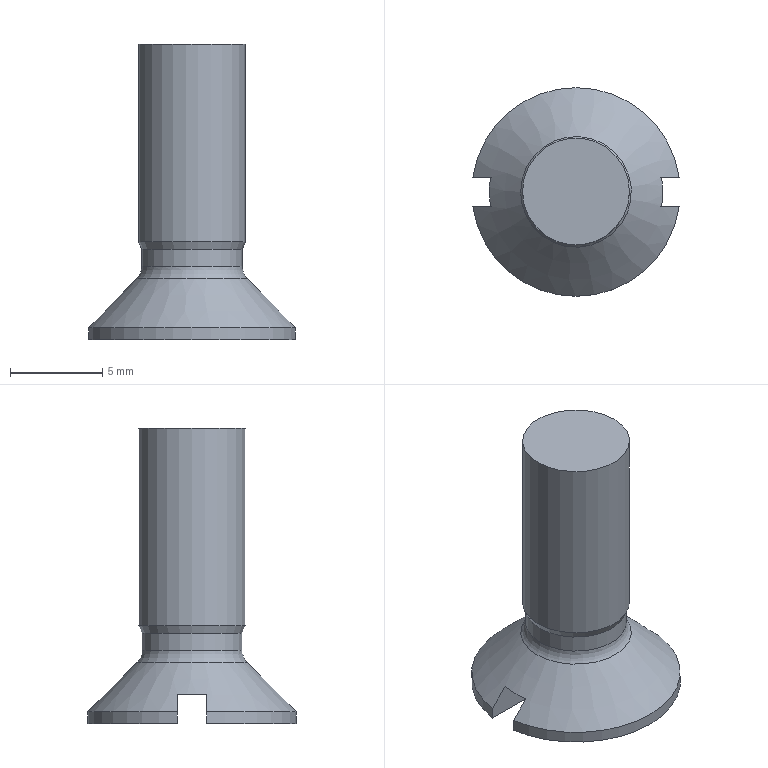Component | NX | GB-T68-2000_M6X16 | 1 solid | 13 faces | box 11.19 x 11.3 x 16 mm | volume 529 mm3 | plane 6 | cylinder 4 | cone 2 | torus 1 | commonest cylinder face diameters 11.3 x2 5.795 x1 5.446 x1
STEP:
#1=CARTESIAN_POINT('',(0.,0.,0.));
#2=DIRECTION('',(0.,0.,1.));
#3=DIRECTION('',(1.,0.,0.));
#4=AXIS2_PLACEMENT_3D('',#1,#2,#3);
#5=CARTESIAN_POINT('',(-384.082,307.381,-745.));
#6=VERTEX_POINT('',#5);
#7=CARTESIAN_POINT('',(-395.268,307.381,-745.));
#8=VERTEX_POINT('',#7);
#9=CARTESIAN_POINT('',(-377.075,307.381,-745.));
#10=DIRECTION('',(-1.,0.,0.));
#11=VECTOR('',#10,1.);
#12=LINE('',#9,#11);
#13=CARTESIAN_POINT('',(-389.675,308.181,-745.));
#14=DIRECTION('',(0.,0.,1.));
#15=DIRECTION('',(-1.,0.,0.));
#16=AXIS2_PLACEMENT_3D('',#13,#14,#15);
#17=PLANE('',#16);
#18=CARTESIAN_POINT('',(-12.6,0.8));
#19=DIRECTION('',(1.,0.));
#20=VECTOR('',#19,1.);
#21=LINE('',#18,#20);
#22=(GEOMETRIC_REPRESENTATION_CONTEXT(2)PARAMETRIC_REPRESENTATION_CONTEXT()REPRESENTATION_CONTEXT('',''));
#23=DEFINITIONAL_REPRESENTATION('',(#21),#22);
#24=PCURVE('',#17,#23);
#25=CARTESIAN_POINT('',(-377.075,307.381,-745.));
#26=DIRECTION('',(0.,-1.,-0.));
#27=DIRECTION('',(0.,0.,-1.));
#28=AXIS2_PLACEMENT_3D('',#25,#26,#27);
#29=PLANE('',#28);
#30=CARTESIAN_POINT('',(0.,0.));
#31=DIRECTION('',(0.,-1.));
#32=VECTOR('',#31,1.);
#33=LINE('',#30,#32);
#34=(GEOMETRIC_REPRESENTATION_CONTEXT(2)PARAMETRIC_REPRESENTATION_CONTEXT()REPRESENTATION_CONTEXT('',''));
#35=DEFINITIONAL_REPRESENTATION('',(#33),#34);
#36=PCURVE('',#29,#35);
#37=SURFACE_CURVE('',#12,(#24,#36),.PCURVE_S1.);
#38=EDGE_CURVE('',#6,#8,#37,.T.);
#39=ORIENTED_EDGE('',*,*,#38,.F.);
#40=CARTESIAN_POINT('',(-389.675,308.181,-745.));
#41=DIRECTION('',(0.,0.,1.));
#42=DIRECTION('',(-1.,0.,0.));
#43=AXIS2_PLACEMENT_3D('',#40,#41,#42);
#44=CIRCLE('',#43,5.65);
#45=CARTESIAN_POINT('',(0.,0.));
#46=DIRECTION('',(1.,0.));
#47=AXIS2_PLACEMENT_2D('',#45,#46);
#48=CIRCLE('',#47,5.65);
#49=(GEOMETRIC_REPRESENTATION_CONTEXT(2)PARAMETRIC_REPRESENTATION_CONTEXT()REPRESENTATION_CONTEXT('',''));
#50=DEFINITIONAL_REPRESENTATION('',(#48),#49);
#51=PCURVE('',#17,#50);
#52=CARTESIAN_POINT('',(-389.675,308.181,-745.));
#53=DIRECTION('',(0.,0.,1.));
#54=DIRECTION('',(-1.,0.,0.));
#55=AXIS2_PLACEMENT_3D('',#52,#53,#54);
#56=CYLINDRICAL_SURFACE('',#55,5.65);
#57=CARTESIAN_POINT('',(0.,0.));
#58=DIRECTION('',(1.,0.));
#59=VECTOR('',#58,1.);
#60=LINE('',#57,#59);
#61=(GEOMETRIC_REPRESENTATION_CONTEXT(2)PARAMETRIC_REPRESENTATION_CONTEXT()REPRESENTATION_CONTEXT('',''));
#62=DEFINITIONAL_REPRESENTATION('',(#60),#61);
#63=PCURVE('',#56,#62);
#64=SURFACE_CURVE('',#44,(#51,#63),.PCURVE_S1.);
#65=EDGE_CURVE('',#8,#6,#64,.T.);
#66=ORIENTED_EDGE('',*,*,#65,.F.);
#67=EDGE_LOOP('',(#39,#66));
#68=FACE_BOUND('',#67,.T.);
#69=ADVANCED_FACE('',(#68),#17,.F.);
#70=ORIENTED_EDGE('',*,*,#65,.T.);
#71=CARTESIAN_POINT('',(-384.082,307.381,-744.35));
#72=VERTEX_POINT('',#71);
#73=CARTESIAN_POINT('',(-384.082,307.381,-745.));
#74=DIRECTION('',(0.,0.,1.));
#75=VECTOR('',#74,1.);
#76=LINE('',#73,#75);
#77=CARTESIAN_POINT('',(3.,0.));
#78=DIRECTION('',(0.,1.));
#79=VECTOR('',#78,1.);
#80=LINE('',#77,#79);
#81=(GEOMETRIC_REPRESENTATION_CONTEXT(2)PARAMETRIC_REPRESENTATION_CONTEXT()REPRESENTATION_CONTEXT('',''));
#82=DEFINITIONAL_REPRESENTATION('',(#80),#81);
#83=PCURVE('',#56,#82);
#84=CARTESIAN_POINT('',(0.,-7.007));
#85=DIRECTION('',(-1.,0.));
#86=VECTOR('',#85,1.);
#87=LINE('',#84,#86);
#88=(GEOMETRIC_REPRESENTATION_CONTEXT(2)PARAMETRIC_REPRESENTATION_CONTEXT()REPRESENTATION_CONTEXT('',''));
#89=DEFINITIONAL_REPRESENTATION('',(#87),#88);
#90=PCURVE('',#29,#89);
#91=SURFACE_CURVE('',#76,(#83,#90),.PCURVE_S1.);
#92=EDGE_CURVE('',#6,#72,#91,.T.);
#93=ORIENTED_EDGE('',*,*,#92,.T.);
#94=CARTESIAN_POINT('',(-395.268,307.381,-744.35));
#95=VERTEX_POINT('',#94);
#96=CARTESIAN_POINT('',(-389.675,308.181,-744.35));
#97=DIRECTION('',(0.,0.,1.));
#98=DIRECTION('',(-1.,0.,0.));
#99=AXIS2_PLACEMENT_3D('',#96,#97,#98);
#100=CIRCLE('',#99,5.65);
#101=CARTESIAN_POINT('',(0.,0.65));
#102=DIRECTION('',(1.,0.));
#103=VECTOR('',#102,1.);
#104=LINE('',#101,#103);
#105=(GEOMETRIC_REPRESENTATION_CONTEXT(2)PARAMETRIC_REPRESENTATION_CONTEXT()REPRESENTATION_CONTEXT('',''));
#106=DEFINITIONAL_REPRESENTATION('',(#104),#105);
#107=PCURVE('',#56,#106);
#108=CARTESIAN_POINT('',(-389.675,308.181,-744.35));
#109=DIRECTION('',(0.,0.,-1.));
#110=DIRECTION('',(1.,0.,0.));
#111=AXIS2_PLACEMENT_3D('',#108,#109,#110);
#112=CONICAL_SURFACE('',#111,5.65,0.7854);
#113=CARTESIAN_POINT('',(3.142,0.));
#114=DIRECTION('',(-1.,0.));
#115=VECTOR('',#114,1.);
#116=LINE('',#113,#115);
#117=(GEOMETRIC_REPRESENTATION_CONTEXT(2)PARAMETRIC_REPRESENTATION_CONTEXT()REPRESENTATION_CONTEXT('',''));
#118=DEFINITIONAL_REPRESENTATION('',(#116),#117);
#119=PCURVE('',#112,#118);
#120=SURFACE_CURVE('',#100,(#107,#119),.PCURVE_S1.);
#121=EDGE_CURVE('',#95,#72,#120,.T.);
#122=ORIENTED_EDGE('',*,*,#121,.F.);
#123=CARTESIAN_POINT('',(-395.268,307.381,-745.));
#124=DIRECTION('',(0.,0.,-1.));
#125=VECTOR('',#124,1.);
#126=LINE('',#123,#125);
#127=CARTESIAN_POINT('',(0.1421,0.));
#128=DIRECTION('',(0.,-1.));
#129=VECTOR('',#128,1.);
#130=LINE('',#127,#129);
#131=(GEOMETRIC_REPRESENTATION_CONTEXT(2)PARAMETRIC_REPRESENTATION_CONTEXT()REPRESENTATION_CONTEXT('',''));
#132=DEFINITIONAL_REPRESENTATION('',(#130),#131);
#133=PCURVE('',#56,#132);
#134=CARTESIAN_POINT('',(0.,-18.193));
#135=DIRECTION('',(1.,0.));
#136=VECTOR('',#135,1.);
#137=LINE('',#134,#136);
#138=(GEOMETRIC_REPRESENTATION_CONTEXT(2)PARAMETRIC_REPRESENTATION_CONTEXT()REPRESENTATION_CONTEXT('',''));
#139=DEFINITIONAL_REPRESENTATION('',(#137),#138);
#140=PCURVE('',#29,#139);
#141=SURFACE_CURVE('',#126,(#133,#140),.PCURVE_S1.);
#142=EDGE_CURVE('',#95,#8,#141,.T.);
#143=ORIENTED_EDGE('',*,*,#142,.T.);
#144=EDGE_LOOP('',(#70,#93,#122,#143));
#145=FACE_BOUND('',#144,.T.);
#146=ADVANCED_FACE('',(#145),#56,.T.);
#147=CARTESIAN_POINT('',(-392.573,308.181,-739.7));
#148=VERTEX_POINT('',#147);
#149=CARTESIAN_POINT('',(-389.675,308.181,-739.7));
#150=DIRECTION('',(0.,0.,1.));
#151=DIRECTION('',(-1.,0.,0.));
#152=AXIS2_PLACEMENT_3D('',#149,#150,#151);
#153=CIRCLE('',#152,2.897);
#154=CARTESIAN_POINT('',(-389.675,308.181,-740.1));
#155=DIRECTION('',(0.,0.,1.));
#156=DIRECTION('',(-1.,0.,0.));
#157=AXIS2_PLACEMENT_3D('',#154,#155,#156);
#158=CONICAL_SURFACE('',#157,2.723,0.4119);
#159=CARTESIAN_POINT('',(0.,0.4));
#160=DIRECTION('',(1.,0.));
#161=VECTOR('',#160,1.);
#162=LINE('',#159,#161);
#163=(GEOMETRIC_REPRESENTATION_CONTEXT(2)PARAMETRIC_REPRESENTATION_CONTEXT()REPRESENTATION_CONTEXT('',''));
#164=DEFINITIONAL_REPRESENTATION('',(#162),#163);
#165=PCURVE('',#158,#164);
#166=CARTESIAN_POINT('',(-389.675,308.181,-745.));
#167=DIRECTION('',(0.,0.,1.));
#168=DIRECTION('',(-1.,0.,0.));
#169=AXIS2_PLACEMENT_3D('',#166,#167,#168);
#170=CYLINDRICAL_SURFACE('',#169,2.897);
#171=CARTESIAN_POINT('',(0.,5.3));
#172=DIRECTION('',(1.,0.));
#173=VECTOR('',#172,1.);
#174=LINE('',#171,#173);
#175=(GEOMETRIC_REPRESENTATION_CONTEXT(2)PARAMETRIC_REPRESENTATION_CONTEXT()REPRESENTATION_CONTEXT('',''));
#176=DEFINITIONAL_REPRESENTATION('',(#174),#175);
#177=PCURVE('',#170,#176);
#178=SURFACE_CURVE('',#153,(#165,#177),.PCURVE_S1.);
#179=EDGE_CURVE('',#148,#148,#178,.T.);
#180=ORIENTED_EDGE('',*,*,#179,.F.);
#181=CARTESIAN_POINT('',(-392.398,308.181,-740.1));
#182=VERTEX_POINT('',#181);
#183=CARTESIAN_POINT('',(-392.398,308.181,-740.1));
#184=CARTESIAN_POINT('',(-392.573,308.181,-739.7));
#185=B_SPLINE_CURVE_WITH_KNOTS('',1,(#183,#184),.UNSPECIFIED.,.F.,.F.,(2,2),(0.,0.4365),.PIECEWISE_BEZIER_KNOTS.);
#186=CARTESIAN_POINT('',(0.,0.));
#187=DIRECTION('',(0.,1.));
#188=VECTOR('',#187,1.);
#189=LINE('',#186,#188);
#190=(GEOMETRIC_REPRESENTATION_CONTEXT(2)PARAMETRIC_REPRESENTATION_CONTEXT()REPRESENTATION_CONTEXT('',''));
#191=DEFINITIONAL_REPRESENTATION('',(#189),#190);
#192=PCURVE('',#158,#191);
#193=CARTESIAN_POINT('',(6.283,0.));
#194=DIRECTION('',(0.,1.));
#195=VECTOR('',#194,1.);
#196=LINE('',#193,#195);
#197=(GEOMETRIC_REPRESENTATION_CONTEXT(2)PARAMETRIC_REPRESENTATION_CONTEXT()REPRESENTATION_CONTEXT('',''));
#198=DEFINITIONAL_REPRESENTATION('',(#196),#197);
#199=PCURVE('',#158,#198);
#200=SEAM_CURVE('',#185,(#192,#199),.PCURVE_S1.);
#201=EDGE_CURVE('',#182,#148,#200,.T.);
#202=ORIENTED_EDGE('',*,*,#201,.F.);
#203=CARTESIAN_POINT('',(-389.675,308.181,-740.1));
#204=DIRECTION('',(0.,0.,1.));
#205=DIRECTION('',(-1.,0.,0.));
#206=AXIS2_PLACEMENT_3D('',#203,#204,#205);
#207=CIRCLE('',#206,2.723);
#208=CARTESIAN_POINT('',(0.,0.));
#209=DIRECTION('',(1.,0.));
#210=VECTOR('',#209,1.);
#211=LINE('',#208,#210);
#212=(GEOMETRIC_REPRESENTATION_CONTEXT(2)PARAMETRIC_REPRESENTATION_CONTEXT()REPRESENTATION_CONTEXT('',''));
#213=DEFINITIONAL_REPRESENTATION('',(#211),#212);
#214=PCURVE('',#158,#213);
#215=CARTESIAN_POINT('',(-389.675,308.181,-745.));
#216=DIRECTION('',(0.,0.,1.));
#217=DIRECTION('',(-1.,0.,0.));
#218=AXIS2_PLACEMENT_3D('',#215,#216,#217);
#219=CYLINDRICAL_SURFACE('',#218,2.723);
#220=CARTESIAN_POINT('',(0.,4.9));
#221=DIRECTION('',(1.,0.));
#222=VECTOR('',#221,1.);
#223=LINE('',#220,#222);
#224=(GEOMETRIC_REPRESENTATION_CONTEXT(2)PARAMETRIC_REPRESENTATION_CONTEXT()REPRESENTATION_CONTEXT('',''));
#225=DEFINITIONAL_REPRESENTATION('',(#223),#224);
#226=PCURVE('',#219,#225);
#227=SURFACE_CURVE('',#207,(#214,#226),.PCURVE_S1.);
#228=EDGE_CURVE('',#182,#182,#227,.T.);
#229=ORIENTED_EDGE('',*,*,#228,.T.);
#230=ORIENTED_EDGE('',*,*,#201,.T.);
#231=EDGE_LOOP('',(#180,#202,#229,#230));
#232=FACE_BOUND('',#231,.T.);
#233=ADVANCED_FACE('',(#232),#158,.T.);
#234=CARTESIAN_POINT('',(-392.573,308.181,-729.));
#235=VERTEX_POINT('',#234);
#236=CARTESIAN_POINT('',(-389.675,308.181,-729.));
#237=DIRECTION('',(0.,0.,1.));
#238=DIRECTION('',(-1.,0.,0.));
#239=AXIS2_PLACEMENT_3D('',#236,#237,#238);
#240=CIRCLE('',#239,2.897);
#241=CARTESIAN_POINT('',(0.,16.));
#242=DIRECTION('',(1.,0.));
#243=VECTOR('',#242,1.);
#244=LINE('',#241,#243);
#245=(GEOMETRIC_REPRESENTATION_CONTEXT(2)PARAMETRIC_REPRESENTATION_CONTEXT()REPRESENTATION_CONTEXT('',''));
#246=DEFINITIONAL_REPRESENTATION('',(#244),#245);
#247=PCURVE('',#170,#246);
#248=CARTESIAN_POINT('',(-389.675,305.284,-729.));
#249=DIRECTION('',(0.,0.,-1.));
#250=DIRECTION('',(1.,0.,0.));
#251=AXIS2_PLACEMENT_3D('',#248,#249,#250);
#252=PLANE('',#251);
#253=CARTESIAN_POINT('',(-2.897,-2.897));
#254=CARTESIAN_POINT('',(-2.897,2.121));
#255=CARTESIAN_POINT('',(1.449,-0.3882));
#256=CARTESIAN_POINT('',(5.795,-2.897));
#257=CARTESIAN_POINT('',(1.449,-5.407));
#258=CARTESIAN_POINT('',(-2.897,-7.916));
#259=CARTESIAN_POINT('',(-2.897,-2.897));
#260=(BOUNDED_CURVE()B_SPLINE_CURVE(2,(#253,#254,#255,#256,#257,#258,#259),.UNSPECIFIED.,.T.,.F.)B_SPLINE_CURVE_WITH_KNOTS((1,2,2,2,2,1),(-2.094,0.,2.094,4.189,6.283,8.378),.UNSPECIFIED.)CURVE()GEOMETRIC_REPRESENTATION_ITEM()RATIONAL_B_SPLINE_CURVE((1.,0.5,1.,0.5,1.,0.5,1.))REPRESENTATION_ITEM(''));
#261=(GEOMETRIC_REPRESENTATION_CONTEXT(2)PARAMETRIC_REPRESENTATION_CONTEXT()REPRESENTATION_CONTEXT('',''));
#262=DEFINITIONAL_REPRESENTATION('',(#260),#261);
#263=PCURVE('',#252,#262);
#264=SURFACE_CURVE('',#240,(#247,#263),.PCURVE_S1.);
#265=EDGE_CURVE('',#235,#235,#264,.T.);
#266=ORIENTED_EDGE('',*,*,#265,.F.);
#267=CARTESIAN_POINT('',(-392.573,308.181,-739.7));
#268=CARTESIAN_POINT('',(-392.573,308.181,-729.));
#269=B_SPLINE_CURVE_WITH_KNOTS('',1,(#267,#268),.UNSPECIFIED.,.F.,.F.,(2,2),(5.3,16.),.PIECEWISE_BEZIER_KNOTS.);
#270=CARTESIAN_POINT('',(0.,0.));
#271=DIRECTION('',(0.,1.));
#272=VECTOR('',#271,1.);
#273=LINE('',#270,#272);
#274=(GEOMETRIC_REPRESENTATION_CONTEXT(2)PARAMETRIC_REPRESENTATION_CONTEXT()REPRESENTATION_CONTEXT('',''));
#275=DEFINITIONAL_REPRESENTATION('',(#273),#274);
#276=PCURVE('',#170,#275);
#277=CARTESIAN_POINT('',(6.283,0.));
#278=DIRECTION('',(0.,1.));
#279=VECTOR('',#278,1.);
#280=LINE('',#277,#279);
#281=(GEOMETRIC_REPRESENTATION_CONTEXT(2)PARAMETRIC_REPRESENTATION_CONTEXT()REPRESENTATION_CONTEXT('',''));
#282=DEFINITIONAL_REPRESENTATION('',(#280),#281);
#283=PCURVE('',#170,#282);
#284=SEAM_CURVE('',#269,(#276,#283),.PCURVE_S1.);
#285=EDGE_CURVE('',#148,#235,#284,.T.);
#286=ORIENTED_EDGE('',*,*,#285,.F.);
#287=ORIENTED_EDGE('',*,*,#179,.T.);
#288=ORIENTED_EDGE('',*,*,#285,.T.);
#289=EDGE_LOOP('',(#266,#286,#287,#288));
#290=FACE_BOUND('',#289,.T.);
#291=ADVANCED_FACE('',(#290),#170,.T.);
#292=ORIENTED_EDGE('',*,*,#265,.T.);
#293=EDGE_LOOP('',(#292));
#294=FACE_BOUND('',#293,.T.);
#295=ADVANCED_FACE('',(#294),#252,.F.);
#296=CARTESIAN_POINT('',(-384.082,308.981,-745.));
#297=VERTEX_POINT('',#296);
#298=CARTESIAN_POINT('',(-395.268,308.981,-745.));
#299=VERTEX_POINT('',#298);
#300=CARTESIAN_POINT('',(-389.675,308.181,-745.));
#301=DIRECTION('',(0.,0.,1.));
#302=DIRECTION('',(-1.,0.,0.));
#303=AXIS2_PLACEMENT_3D('',#300,#301,#302);
#304=CIRCLE('',#303,5.65);
#305=CARTESIAN_POINT('',(-389.675,308.181,-745.));
#306=DIRECTION('',(0.,0.,1.));
#307=DIRECTION('',(-1.,0.,0.));
#308=AXIS2_PLACEMENT_3D('',#305,#306,#307);
#309=PLANE('',#308);
#310=CARTESIAN_POINT('',(0.,0.));
#311=DIRECTION('',(1.,0.));
#312=AXIS2_PLACEMENT_2D('',#310,#311);
#313=CIRCLE('',#312,5.65);
#314=(GEOMETRIC_REPRESENTATION_CONTEXT(2)PARAMETRIC_REPRESENTATION_CONTEXT()REPRESENTATION_CONTEXT('',''));
#315=DEFINITIONAL_REPRESENTATION('',(#313),#314);
#316=PCURVE('',#309,#315);
#317=CARTESIAN_POINT('',(-389.675,308.181,-745.));
#318=DIRECTION('',(0.,0.,1.));
#319=DIRECTION('',(-1.,0.,0.));
#320=AXIS2_PLACEMENT_3D('',#317,#318,#319);
#321=CYLINDRICAL_SURFACE('',#320,5.65);
#322=CARTESIAN_POINT('',(0.,0.));
#323=DIRECTION('',(1.,0.));
#324=VECTOR('',#323,1.);
#325=LINE('',#322,#324);
#326=(GEOMETRIC_REPRESENTATION_CONTEXT(2)PARAMETRIC_REPRESENTATION_CONTEXT()REPRESENTATION_CONTEXT('',''));
#327=DEFINITIONAL_REPRESENTATION('',(#325),#326);
#328=PCURVE('',#321,#327);
#329=SURFACE_CURVE('',#304,(#316,#328),.PCURVE_S1.);
#330=EDGE_CURVE('',#297,#299,#329,.T.);
#331=ORIENTED_EDGE('',*,*,#330,.F.);
#332=CARTESIAN_POINT('',(-377.075,308.981,-745.));
#333=DIRECTION('',(-1.,0.,0.));
#334=VECTOR('',#333,1.);
#335=LINE('',#332,#334);
#336=CARTESIAN_POINT('',(-12.6,-0.8));
#337=DIRECTION('',(1.,0.));
#338=VECTOR('',#337,1.);
#339=LINE('',#336,#338);
#340=(GEOMETRIC_REPRESENTATION_CONTEXT(2)PARAMETRIC_REPRESENTATION_CONTEXT()REPRESENTATION_CONTEXT('',''));
#341=DEFINITIONAL_REPRESENTATION('',(#339),#340);
#342=PCURVE('',#309,#341);
#343=CARTESIAN_POINT('',(-377.075,308.981,-743.4));
#344=DIRECTION('',(0.,1.,0.));
#345=DIRECTION('',(0.,-0.,1.));
#346=AXIS2_PLACEMENT_3D('',#343,#344,#345);
#347=PLANE('',#346);
#348=CARTESIAN_POINT('',(-1.6,0.));
#349=DIRECTION('',(0.,-1.));
#350=VECTOR('',#349,1.);
#351=LINE('',#348,#350);
#352=(GEOMETRIC_REPRESENTATION_CONTEXT(2)PARAMETRIC_REPRESENTATION_CONTEXT()REPRESENTATION_CONTEXT('',''));
#353=DEFINITIONAL_REPRESENTATION('',(#351),#352);
#354=PCURVE('',#347,#353);
#355=SURFACE_CURVE('',#335,(#342,#354),.PCURVE_S1.);
#356=EDGE_CURVE('',#297,#299,#355,.T.);
#357=ORIENTED_EDGE('',*,*,#356,.T.);
#358=EDGE_LOOP('',(#331,#357));
#359=FACE_BOUND('',#358,.T.);
#360=ADVANCED_FACE('',(#359),#309,.F.);
#361=ORIENTED_EDGE('',*,*,#330,.T.);
#362=CARTESIAN_POINT('',(-395.268,308.981,-744.35));
#363=VERTEX_POINT('',#362);
#364=CARTESIAN_POINT('',(-395.268,308.981,-745.));
#365=DIRECTION('',(0.,0.,1.));
#366=VECTOR('',#365,1.);
#367=LINE('',#364,#366);
#368=CARTESIAN_POINT('',(6.141,0.));
#369=DIRECTION('',(0.,1.));
#370=VECTOR('',#369,1.);
#371=LINE('',#368,#370);
#372=(GEOMETRIC_REPRESENTATION_CONTEXT(2)PARAMETRIC_REPRESENTATION_CONTEXT()REPRESENTATION_CONTEXT('',''));
#373=DEFINITIONAL_REPRESENTATION('',(#371),#372);
#374=PCURVE('',#321,#373);
#375=CARTESIAN_POINT('',(-1.6,-18.193));
#376=DIRECTION('',(1.,0.));
#377=VECTOR('',#376,1.);
#378=LINE('',#375,#377);
#379=(GEOMETRIC_REPRESENTATION_CONTEXT(2)PARAMETRIC_REPRESENTATION_CONTEXT()REPRESENTATION_CONTEXT('',''));
#380=DEFINITIONAL_REPRESENTATION('',(#378),#379);
#381=PCURVE('',#347,#380);
#382=SURFACE_CURVE('',#367,(#374,#381),.PCURVE_S1.);
#383=EDGE_CURVE('',#299,#363,#382,.T.);
#384=ORIENTED_EDGE('',*,*,#383,.T.);
#385=CARTESIAN_POINT('',(-384.082,308.981,-744.35));
#386=VERTEX_POINT('',#385);
#387=CARTESIAN_POINT('',(-389.675,308.181,-744.35));
#388=DIRECTION('',(0.,0.,1.));
#389=DIRECTION('',(-1.,0.,0.));
#390=AXIS2_PLACEMENT_3D('',#387,#388,#389);
#391=CIRCLE('',#390,5.65);
#392=CARTESIAN_POINT('',(0.,0.65));
#393=DIRECTION('',(1.,0.));
#394=VECTOR('',#393,1.);
#395=LINE('',#392,#394);
#396=(GEOMETRIC_REPRESENTATION_CONTEXT(2)PARAMETRIC_REPRESENTATION_CONTEXT()REPRESENTATION_CONTEXT('',''));
#397=DEFINITIONAL_REPRESENTATION('',(#395),#396);
#398=PCURVE('',#321,#397);
#399=CARTESIAN_POINT('',(9.425,0.));
#400=DIRECTION('',(-1.,0.));
#401=VECTOR('',#400,1.);
#402=LINE('',#399,#401);
#403=(GEOMETRIC_REPRESENTATION_CONTEXT(2)PARAMETRIC_REPRESENTATION_CONTEXT()REPRESENTATION_CONTEXT('',''));
#404=DEFINITIONAL_REPRESENTATION('',(#402),#403);
#405=PCURVE('',#112,#404);
#406=SURFACE_CURVE('',#391,(#398,#405),.PCURVE_S1.);
#407=EDGE_CURVE('',#386,#363,#406,.T.);
#408=ORIENTED_EDGE('',*,*,#407,.F.);
#409=CARTESIAN_POINT('',(-384.082,308.981,-745.));
#410=DIRECTION('',(0.,0.,-1.));
#411=VECTOR('',#410,1.);
#412=LINE('',#409,#411);
#413=CARTESIAN_POINT('',(3.284,0.));
#414=DIRECTION('',(0.,-1.));
#415=VECTOR('',#414,1.);
#416=LINE('',#413,#415);
#417=(GEOMETRIC_REPRESENTATION_CONTEXT(2)PARAMETRIC_REPRESENTATION_CONTEXT()REPRESENTATION_CONTEXT('',''));
#418=DEFINITIONAL_REPRESENTATION('',(#416),#417);
#419=PCURVE('',#321,#418);
#420=CARTESIAN_POINT('',(-1.6,-7.007));
#421=DIRECTION('',(-1.,0.));
#422=VECTOR('',#421,1.);
#423=LINE('',#420,#422);
#424=(GEOMETRIC_REPRESENTATION_CONTEXT(2)PARAMETRIC_REPRESENTATION_CONTEXT()REPRESENTATION_CONTEXT('',''));
#425=DEFINITIONAL_REPRESENTATION('',(#423),#424);
#426=PCURVE('',#347,#425);
#427=SURFACE_CURVE('',#412,(#419,#426),.PCURVE_S1.);
#428=EDGE_CURVE('',#386,#297,#427,.T.);
#429=ORIENTED_EDGE('',*,*,#428,.T.);
#430=EDGE_LOOP('',(#361,#384,#408,#429));
#431=FACE_BOUND('',#430,.T.);
#432=ADVANCED_FACE('',(#431),#321,.T.);
#433=CARTESIAN_POINT('',(-386.706,307.757,-741.7));
#434=VERTEX_POINT('',#433);
#435=CARTESIAN_POINT('',(-392.675,308.181,-741.7));
#436=VERTEX_POINT('',#435);
#437=CARTESIAN_POINT('',(-389.675,308.181,-741.7));
#438=DIRECTION('',(0.,0.,1.));
#439=DIRECTION('',(-1.,0.,0.));
#440=AXIS2_PLACEMENT_3D('',#437,#438,#439);
#441=CIRCLE('',#440,3.);
#442=CARTESIAN_POINT('',(9.425,-2.65));
#443=DIRECTION('',(-1.,0.));
#444=VECTOR('',#443,1.);
#445=LINE('',#442,#444);
#446=(GEOMETRIC_REPRESENTATION_CONTEXT(2)PARAMETRIC_REPRESENTATION_CONTEXT()REPRESENTATION_CONTEXT('',''));
#447=DEFINITIONAL_REPRESENTATION('',(#445),#446);
#448=PCURVE('',#112,#447);
#449=CARTESIAN_POINT('',(-389.675,308.181,-741.031));
#450=DIRECTION('',(0.,0.,1.));
#451=DIRECTION('',(-1.,0.,0.));
#452=AXIS2_PLACEMENT_3D('',#449,#450,#451);
#453=TOROIDAL_SURFACE('',#452,3.669,0.9466);
#454=CARTESIAN_POINT('',(0.,3.927));
#455=DIRECTION('',(1.,-0.));
#456=VECTOR('',#455,1.);
#457=LINE('',#454,#456);
#458=(GEOMETRIC_REPRESENTATION_CONTEXT(2)PARAMETRIC_REPRESENTATION_CONTEXT()REPRESENTATION_CONTEXT('',''));
#459=DEFINITIONAL_REPRESENTATION('',(#457),#458);
#460=PCURVE('',#453,#459);
#461=SURFACE_CURVE('',#441,(#448,#460),.PCURVE_S1.);
#462=EDGE_CURVE('',#434,#436,#461,.T.);
#463=ORIENTED_EDGE('',*,*,#462,.F.);
#464=CARTESIAN_POINT('',(-385.023,307.516,-743.4));
#465=VERTEX_POINT('',#464);
#466=CARTESIAN_POINT('',(-386.706,307.757,-741.7));
#467=CARTESIAN_POINT('',(-385.023,307.516,-743.4));
#468=B_SPLINE_CURVE_WITH_KNOTS('',1,(#466,#467),.UNSPECIFIED.,.F.,.F.,(2,2),(-3.748,-1.344),.PIECEWISE_BEZIER_KNOTS.);
#469=CARTESIAN_POINT('',(6.425,0.));
#470=DIRECTION('',(0.,1.));
#471=VECTOR('',#470,1.);
#472=LINE('',#469,#471);
#473=(GEOMETRIC_REPRESENTATION_CONTEXT(2)PARAMETRIC_REPRESENTATION_CONTEXT()REPRESENTATION_CONTEXT('',''));
#474=DEFINITIONAL_REPRESENTATION('',(#472),#473);
#475=PCURVE('',#112,#474);
#476=CARTESIAN_POINT('',(0.1421,0.));
#477=DIRECTION('',(0.,1.));
#478=VECTOR('',#477,1.);
#479=LINE('',#476,#478);
#480=(GEOMETRIC_REPRESENTATION_CONTEXT(2)PARAMETRIC_REPRESENTATION_CONTEXT()REPRESENTATION_CONTEXT('',''));
#481=DEFINITIONAL_REPRESENTATION('',(#479),#480);
#482=PCURVE('',#112,#481);
#483=SEAM_CURVE('',#468,(#475,#482),.PCURVE_S1.);
#484=EDGE_CURVE('',#434,#465,#483,.T.);
#485=ORIENTED_EDGE('',*,*,#484,.T.);
#486=CARTESIAN_POINT('',(-385.044,308.981,-743.4));
#487=VERTEX_POINT('',#486);
#488=CARTESIAN_POINT('',(-389.675,308.181,-743.4));
#489=DIRECTION('',(0.,0.,1.));
#490=DIRECTION('',(-1.,0.,0.));
#491=AXIS2_PLACEMENT_3D('',#488,#489,#490);
#492=CIRCLE('',#491,4.7);
#493=CARTESIAN_POINT('',(9.425,-0.95));
#494=DIRECTION('',(-1.,0.));
#495=VECTOR('',#494,1.);
#496=LINE('',#493,#495);
#497=(GEOMETRIC_REPRESENTATION_CONTEXT(2)PARAMETRIC_REPRESENTATION_CONTEXT()REPRESENTATION_CONTEXT('',''));
#498=DEFINITIONAL_REPRESENTATION('',(#496),#497);
#499=PCURVE('',#112,#498);
#500=CARTESIAN_POINT('',(-377.075,308.181,-743.4));
#501=DIRECTION('',(0.,0.,1.));
#502=DIRECTION('',(-1.,0.,0.));
#503=AXIS2_PLACEMENT_3D('',#500,#501,#502);
#504=PLANE('',#503);
#505=CARTESIAN_POINT('',(12.6,0.));
#506=DIRECTION('',(1.,0.));
#507=AXIS2_PLACEMENT_2D('',#505,#506);
#508=CIRCLE('',#507,4.7);
#509=(GEOMETRIC_REPRESENTATION_CONTEXT(2)PARAMETRIC_REPRESENTATION_CONTEXT()REPRESENTATION_CONTEXT('',''));
#510=DEFINITIONAL_REPRESENTATION('',(#508),#509);
#511=PCURVE('',#504,#510);
#512=SURFACE_CURVE('',#492,(#499,#511),.PCURVE_S1.);
#513=EDGE_CURVE('',#465,#487,#512,.T.);
#514=ORIENTED_EDGE('',*,*,#513,.T.);
#515=CARTESIAN_POINT('',(-385.044,308.981,-743.4));
#516=CARTESIAN_POINT('',(-384.723,308.981,-743.716));
#517=CARTESIAN_POINT('',(-384.402,308.981,-744.033));
#518=CARTESIAN_POINT('',(-384.082,308.981,-744.35));
#519=B_SPLINE_CURVE_WITH_KNOTS('',3,(#515,#516,#517,#518),.UNSPECIFIED.,.F.,.F.,(4,4),(0.,1.),.PIECEWISE_BEZIER_KNOTS.);
#520=CARTESIAN_POINT('',(6.112,-0.95));
#521=CARTESIAN_POINT('',(6.141,0.));
#522=B_SPLINE_CURVE_WITH_KNOTS('',1,(#520,#521),.UNSPECIFIED.,.F.,.F.,(2,2),(0.,1.),.PIECEWISE_BEZIER_KNOTS.);
#523=(GEOMETRIC_REPRESENTATION_CONTEXT(2)PARAMETRIC_REPRESENTATION_CONTEXT()REPRESENTATION_CONTEXT('',''));
#524=DEFINITIONAL_REPRESENTATION('',(#522),#523);
#525=PCURVE('',#112,#524);
#526=CARTESIAN_POINT('',(0.,-7.969));
#527=CARTESIAN_POINT('',(-0.3163,-7.648));
#528=CARTESIAN_POINT('',(-0.633,-7.327));
#529=CARTESIAN_POINT('',(-0.95,-7.007));
#530=B_SPLINE_CURVE_WITH_KNOTS('',3,(#526,#527,#528,#529),.UNSPECIFIED.,.F.,.F.,(4,4),(0.,1.),.PIECEWISE_BEZIER_KNOTS.);
#531=(GEOMETRIC_REPRESENTATION_CONTEXT(2)PARAMETRIC_REPRESENTATION_CONTEXT()REPRESENTATION_CONTEXT('',''));
#532=DEFINITIONAL_REPRESENTATION('',(#530),#531);
#533=PCURVE('',#347,#532);
#534=SURFACE_CURVE('',#519,(#525,#533),.PCURVE_S1.);
#535=EDGE_CURVE('',#487,#386,#534,.T.);
#536=ORIENTED_EDGE('',*,*,#535,.T.);
#537=ORIENTED_EDGE('',*,*,#407,.T.);
#538=CARTESIAN_POINT('',(-394.307,308.981,-743.4));
#539=VERTEX_POINT('',#538);
#540=CARTESIAN_POINT('',(-395.268,308.981,-744.35));
#541=CARTESIAN_POINT('',(-394.948,308.981,-744.033));
#542=CARTESIAN_POINT('',(-394.628,308.981,-743.716));
#543=CARTESIAN_POINT('',(-394.307,308.981,-743.4));
#544=B_SPLINE_CURVE_WITH_KNOTS('',3,(#540,#541,#542,#543),.UNSPECIFIED.,.F.,.F.,(4,4),(0.,1.),.PIECEWISE_BEZIER_KNOTS.);
#545=CARTESIAN_POINT('',(3.284,0.));
#546=CARTESIAN_POINT('',(3.313,-0.95));
#547=B_SPLINE_CURVE_WITH_KNOTS('',1,(#545,#546),.UNSPECIFIED.,.F.,.F.,(2,2),(0.,1.),.PIECEWISE_BEZIER_KNOTS.);
#548=(GEOMETRIC_REPRESENTATION_CONTEXT(2)PARAMETRIC_REPRESENTATION_CONTEXT()REPRESENTATION_CONTEXT('',''));
#549=DEFINITIONAL_REPRESENTATION('',(#547),#548);
#550=PCURVE('',#112,#549);
#551=CARTESIAN_POINT('',(-0.95,-18.193));
#552=CARTESIAN_POINT('',(-0.633,-17.873));
#553=CARTESIAN_POINT('',(-0.3163,-17.552));
#554=CARTESIAN_POINT('',(0.,-17.231));
#555=B_SPLINE_CURVE_WITH_KNOTS('',3,(#551,#552,#553,#554),.UNSPECIFIED.,.F.,.F.,(4,4),(0.,1.),.PIECEWISE_BEZIER_KNOTS.);
#556=(GEOMETRIC_REPRESENTATION_CONTEXT(2)PARAMETRIC_REPRESENTATION_CONTEXT()REPRESENTATION_CONTEXT('',''));
#557=DEFINITIONAL_REPRESENTATION('',(#555),#556);
#558=PCURVE('',#347,#557);
#559=SURFACE_CURVE('',#544,(#550,#558),.PCURVE_S1.);
#560=EDGE_CURVE('',#363,#539,#559,.T.);
#561=ORIENTED_EDGE('',*,*,#560,.T.);
#562=CARTESIAN_POINT('',(-394.307,307.381,-743.4));
#563=VERTEX_POINT('',#562);
#564=CARTESIAN_POINT('',(-389.675,308.181,-743.4));
#565=DIRECTION('',(0.,0.,1.));
#566=DIRECTION('',(-1.,0.,0.));
#567=AXIS2_PLACEMENT_3D('',#564,#565,#566);
#568=CIRCLE('',#567,4.7);
#569=CARTESIAN_POINT('',(9.425,-0.95));
#570=DIRECTION('',(-1.,0.));
#571=VECTOR('',#570,1.);
#572=LINE('',#569,#571);
#573=(GEOMETRIC_REPRESENTATION_CONTEXT(2)PARAMETRIC_REPRESENTATION_CONTEXT()REPRESENTATION_CONTEXT('',''));
#574=DEFINITIONAL_REPRESENTATION('',(#572),#573);
#575=PCURVE('',#112,#574);
#576=CARTESIAN_POINT('',(12.6,0.));
#577=DIRECTION('',(1.,0.));
#578=AXIS2_PLACEMENT_2D('',#576,#577);
#579=CIRCLE('',#578,4.7);
#580=(GEOMETRIC_REPRESENTATION_CONTEXT(2)PARAMETRIC_REPRESENTATION_CONTEXT()REPRESENTATION_CONTEXT('',''));
#581=DEFINITIONAL_REPRESENTATION('',(#579),#580);
#582=PCURVE('',#504,#581);
#583=SURFACE_CURVE('',#568,(#575,#582),.PCURVE_S1.);
#584=EDGE_CURVE('',#539,#563,#583,.T.);
#585=ORIENTED_EDGE('',*,*,#584,.T.);
#586=CARTESIAN_POINT('',(-394.307,307.381,-743.4));
#587=CARTESIAN_POINT('',(-394.628,307.381,-743.716));
#588=CARTESIAN_POINT('',(-394.948,307.381,-744.033));
#589=CARTESIAN_POINT('',(-395.268,307.381,-744.35));
#590=B_SPLINE_CURVE_WITH_KNOTS('',3,(#586,#587,#588,#589),.UNSPECIFIED.,.F.,.F.,(4,4),(0.,1.),.PIECEWISE_BEZIER_KNOTS.);
#591=CARTESIAN_POINT('',(2.971,-0.95));
#592=CARTESIAN_POINT('',(3.,0.));
#593=B_SPLINE_CURVE_WITH_KNOTS('',1,(#591,#592),.UNSPECIFIED.,.F.,.F.,(2,2),(0.,1.),.PIECEWISE_BEZIER_KNOTS.);
#594=(GEOMETRIC_REPRESENTATION_CONTEXT(2)PARAMETRIC_REPRESENTATION_CONTEXT()REPRESENTATION_CONTEXT('',''));
#595=DEFINITIONAL_REPRESENTATION('',(#593),#594);
#596=PCURVE('',#112,#595);
#597=CARTESIAN_POINT('',(-1.6,-17.231));
#598=CARTESIAN_POINT('',(-1.284,-17.552));
#599=CARTESIAN_POINT('',(-0.967,-17.873));
#600=CARTESIAN_POINT('',(-0.65,-18.193));
#601=B_SPLINE_CURVE_WITH_KNOTS('',3,(#597,#598,#599,#600),.UNSPECIFIED.,.F.,.F.,(4,4),(0.,1.),.PIECEWISE_BEZIER_KNOTS.);
#602=(GEOMETRIC_REPRESENTATION_CONTEXT(2)PARAMETRIC_REPRESENTATION_CONTEXT()REPRESENTATION_CONTEXT('',''));
#603=DEFINITIONAL_REPRESENTATION('',(#601),#602);
#604=PCURVE('',#29,#603);
#605=SURFACE_CURVE('',#590,(#596,#604),.PCURVE_S1.);
#606=EDGE_CURVE('',#563,#95,#605,.T.);
#607=ORIENTED_EDGE('',*,*,#606,.T.);
#608=ORIENTED_EDGE('',*,*,#121,.T.);
#609=CARTESIAN_POINT('',(-385.044,307.381,-743.4));
#610=VERTEX_POINT('',#609);
#611=CARTESIAN_POINT('',(-384.082,307.381,-744.35));
#612=CARTESIAN_POINT('',(-384.402,307.381,-744.033));
#613=CARTESIAN_POINT('',(-384.723,307.381,-743.716));
#614=CARTESIAN_POINT('',(-385.044,307.381,-743.4));
#615=B_SPLINE_CURVE_WITH_KNOTS('',3,(#611,#612,#613,#614),.UNSPECIFIED.,.F.,.F.,(4,4),(0.,1.),.PIECEWISE_BEZIER_KNOTS.);
#616=CARTESIAN_POINT('',(0.1421,0.));
#617=CARTESIAN_POINT('',(0.171,-0.95));
#618=B_SPLINE_CURVE_WITH_KNOTS('',1,(#616,#617),.UNSPECIFIED.,.F.,.F.,(2,2),(0.,1.),.PIECEWISE_BEZIER_KNOTS.);
#619=(GEOMETRIC_REPRESENTATION_CONTEXT(2)PARAMETRIC_REPRESENTATION_CONTEXT()REPRESENTATION_CONTEXT('',''));
#620=DEFINITIONAL_REPRESENTATION('',(#618),#619);
#621=PCURVE('',#112,#620);
#622=CARTESIAN_POINT('',(-0.65,-7.007));
#623=CARTESIAN_POINT('',(-0.967,-7.327));
#624=CARTESIAN_POINT('',(-1.284,-7.648));
#625=CARTESIAN_POINT('',(-1.6,-7.969));
#626=B_SPLINE_CURVE_WITH_KNOTS('',3,(#622,#623,#624,#625),.UNSPECIFIED.,.F.,.F.,(4,4),(0.,1.),.PIECEWISE_BEZIER_KNOTS.);
#627=(GEOMETRIC_REPRESENTATION_CONTEXT(2)PARAMETRIC_REPRESENTATION_CONTEXT()REPRESENTATION_CONTEXT('',''));
#628=DEFINITIONAL_REPRESENTATION('',(#626),#627);
#629=PCURVE('',#29,#628);
#630=SURFACE_CURVE('',#615,(#621,#629),.PCURVE_S1.);
#631=EDGE_CURVE('',#72,#610,#630,.T.);
#632=ORIENTED_EDGE('',*,*,#631,.T.);
#633=CARTESIAN_POINT('',(-389.675,308.181,-743.4));
#634=DIRECTION('',(0.,0.,1.));
#635=DIRECTION('',(-1.,0.,0.));
#636=AXIS2_PLACEMENT_3D('',#633,#634,#635);
#637=CIRCLE('',#636,4.7);
#638=CARTESIAN_POINT('',(3.142,-0.95));
#639=DIRECTION('',(-1.,0.));
#640=VECTOR('',#639,1.);
#641=LINE('',#638,#640);
#642=(GEOMETRIC_REPRESENTATION_CONTEXT(2)PARAMETRIC_REPRESENTATION_CONTEXT()REPRESENTATION_CONTEXT('',''));
#643=DEFINITIONAL_REPRESENTATION('',(#641),#642);
#644=PCURVE('',#112,#643);
#645=CARTESIAN_POINT('',(12.6,0.));
#646=DIRECTION('',(1.,0.));
#647=AXIS2_PLACEMENT_2D('',#645,#646);
#648=CIRCLE('',#647,4.7);
#649=(GEOMETRIC_REPRESENTATION_CONTEXT(2)PARAMETRIC_REPRESENTATION_CONTEXT()REPRESENTATION_CONTEXT('',''));
#650=DEFINITIONAL_REPRESENTATION('',(#648),#649);
#651=PCURVE('',#504,#650);
#652=SURFACE_CURVE('',#637,(#644,#651),.PCURVE_S1.);
#653=EDGE_CURVE('',#610,#465,#652,.T.);
#654=ORIENTED_EDGE('',*,*,#653,.T.);
#655=ORIENTED_EDGE('',*,*,#484,.F.);
#656=CARTESIAN_POINT('',(-389.675,308.181,-741.7));
#657=DIRECTION('',(0.,0.,1.));
#658=DIRECTION('',(-1.,0.,0.));
#659=AXIS2_PLACEMENT_3D('',#656,#657,#658);
#660=CIRCLE('',#659,3.);
#661=CARTESIAN_POINT('',(3.142,-2.65));
#662=DIRECTION('',(-1.,0.));
#663=VECTOR('',#662,1.);
#664=LINE('',#661,#663);
#665=(GEOMETRIC_REPRESENTATION_CONTEXT(2)PARAMETRIC_REPRESENTATION_CONTEXT()REPRESENTATION_CONTEXT('',''));
#666=DEFINITIONAL_REPRESENTATION('',(#664),#665);
#667=PCURVE('',#112,#666);
#668=CARTESIAN_POINT('',(0.,3.927));
#669=DIRECTION('',(1.,0.));
#670=VECTOR('',#669,1.);
#671=LINE('',#668,#670);
#672=(GEOMETRIC_REPRESENTATION_CONTEXT(2)PARAMETRIC_REPRESENTATION_CONTEXT()REPRESENTATION_CONTEXT('',''));
#673=DEFINITIONAL_REPRESENTATION('',(#671),#672);
#674=PCURVE('',#453,#673);
#675=SURFACE_CURVE('',#660,(#667,#674),.PCURVE_S1.);
#676=EDGE_CURVE('',#436,#434,#675,.T.);
#677=ORIENTED_EDGE('',*,*,#676,.F.);
#678=EDGE_LOOP('',(#463,#485,#514,#536,#537,#561,#585,#607,#608,#632,#654,#655,#677));
#679=FACE_BOUND('',#678,.T.);
#680=ADVANCED_FACE('',(#679),#112,.T.);
#681=CARTESIAN_POINT('',(-392.398,308.181,-741.031));
#682=VERTEX_POINT('',#681);
#683=CARTESIAN_POINT('',(-389.675,308.181,-741.031));
#684=DIRECTION('',(0.,0.,1.));
#685=DIRECTION('',(-1.,0.,0.));
#686=AXIS2_PLACEMENT_3D('',#683,#684,#685);
#687=CIRCLE('',#686,2.723);
#688=CARTESIAN_POINT('',(0.,3.142));
#689=DIRECTION('',(1.,0.));
#690=VECTOR('',#689,1.);
#691=LINE('',#688,#690);
#692=(GEOMETRIC_REPRESENTATION_CONTEXT(2)PARAMETRIC_REPRESENTATION_CONTEXT()REPRESENTATION_CONTEXT('',''));
#693=DEFINITIONAL_REPRESENTATION('',(#691),#692);
#694=PCURVE('',#453,#693);
#695=CARTESIAN_POINT('',(0.,3.969));
#696=DIRECTION('',(1.,0.));
#697=VECTOR('',#696,1.);
#698=LINE('',#695,#697);
#699=(GEOMETRIC_REPRESENTATION_CONTEXT(2)PARAMETRIC_REPRESENTATION_CONTEXT()REPRESENTATION_CONTEXT('',''));
#700=DEFINITIONAL_REPRESENTATION('',(#698),#699);
#701=PCURVE('',#219,#700);
#702=SURFACE_CURVE('',#687,(#694,#701),.PCURVE_S1.);
#703=EDGE_CURVE('',#682,#682,#702,.T.);
#704=ORIENTED_EDGE('',*,*,#703,.T.);
#705=CARTESIAN_POINT('',(-392.398,308.181,-741.031));
#706=CARTESIAN_POINT('',(-392.398,308.181,-741.155));
#707=CARTESIAN_POINT('',(-392.418,308.181,-741.279));
#708=CARTESIAN_POINT('',(-392.457,308.181,-741.399));
#709=CARTESIAN_POINT('',(-392.514,308.181,-741.511));
#710=CARTESIAN_POINT('',(-392.587,308.181,-741.612));
#711=CARTESIAN_POINT('',(-392.675,308.181,-741.7));
#712=(BOUNDED_CURVE()B_SPLINE_CURVE(6,(#705,#706,#707,#708,#709,#710,#711),.UNSPECIFIED.,.F.,.F.)B_SPLINE_CURVE_WITH_KNOTS((7,7),(3.142,3.927),.PIECEWISE_BEZIER_KNOTS.)CURVE()GEOMETRIC_REPRESENTATION_ITEM()RATIONAL_B_SPLINE_CURVE((1.008,1.003,0.9995,0.9985,0.9995,1.003,1.008))REPRESENTATION_ITEM(''));
#713=CARTESIAN_POINT('',(6.283,0.));
#714=DIRECTION('',(0.,1.));
#715=VECTOR('',#714,1.);
#716=LINE('',#713,#715);
#717=(GEOMETRIC_REPRESENTATION_CONTEXT(2)PARAMETRIC_REPRESENTATION_CONTEXT()REPRESENTATION_CONTEXT('',''));
#718=DEFINITIONAL_REPRESENTATION('',(#716),#717);
#719=PCURVE('',#453,#718);
#720=CARTESIAN_POINT('',(0.,0.));
#721=DIRECTION('',(0.,1.));
#722=VECTOR('',#721,1.);
#723=LINE('',#720,#722);
#724=(GEOMETRIC_REPRESENTATION_CONTEXT(2)PARAMETRIC_REPRESENTATION_CONTEXT()REPRESENTATION_CONTEXT('',''));
#725=DEFINITIONAL_REPRESENTATION('',(#723),#724);
#726=PCURVE('',#453,#725);
#727=SEAM_CURVE('',#712,(#719,#726),.PCURVE_S1.);
#728=EDGE_CURVE('',#682,#436,#727,.T.);
#729=ORIENTED_EDGE('',*,*,#728,.T.);
#730=ORIENTED_EDGE('',*,*,#462,.F.);
#731=ORIENTED_EDGE('',*,*,#676,.F.);
#732=ORIENTED_EDGE('',*,*,#728,.F.);
#733=EDGE_LOOP('',(#704,#729,#730,#731,#732));
#734=FACE_BOUND('',#733,.F.);
#735=ADVANCED_FACE('',(#734),#453,.F.);
#736=ORIENTED_EDGE('',*,*,#228,.F.);
#737=CARTESIAN_POINT('',(-392.398,308.181,-741.031));
#738=CARTESIAN_POINT('',(-392.398,308.181,-740.1));
#739=B_SPLINE_CURVE_WITH_KNOTS('',1,(#737,#738),.UNSPECIFIED.,.F.,.F.,(2,2),(3.969,4.9),.PIECEWISE_BEZIER_KNOTS.);
#740=CARTESIAN_POINT('',(0.,0.));
#741=DIRECTION('',(0.,1.));
#742=VECTOR('',#741,1.);
#743=LINE('',#740,#742);
#744=(GEOMETRIC_REPRESENTATION_CONTEXT(2)PARAMETRIC_REPRESENTATION_CONTEXT()REPRESENTATION_CONTEXT('',''));
#745=DEFINITIONAL_REPRESENTATION('',(#743),#744);
#746=PCURVE('',#219,#745);
#747=CARTESIAN_POINT('',(6.283,0.));
#748=DIRECTION('',(0.,1.));
#749=VECTOR('',#748,1.);
#750=LINE('',#747,#749);
#751=(GEOMETRIC_REPRESENTATION_CONTEXT(2)PARAMETRIC_REPRESENTATION_CONTEXT()REPRESENTATION_CONTEXT('',''));
#752=DEFINITIONAL_REPRESENTATION('',(#750),#751);
#753=PCURVE('',#219,#752);
#754=SEAM_CURVE('',#739,(#746,#753),.PCURVE_S1.);
#755=EDGE_CURVE('',#682,#182,#754,.T.);
#756=ORIENTED_EDGE('',*,*,#755,.F.);
#757=ORIENTED_EDGE('',*,*,#703,.T.);
#758=ORIENTED_EDGE('',*,*,#755,.T.);
#759=EDGE_LOOP('',(#736,#756,#757,#758));
#760=FACE_BOUND('',#759,.T.);
#761=ADVANCED_FACE('',(#760),#219,.T.);
#762=ORIENTED_EDGE('',*,*,#38,.T.);
#763=ORIENTED_EDGE('',*,*,#142,.F.);
#764=ORIENTED_EDGE('',*,*,#606,.F.);
#765=CARTESIAN_POINT('',(-377.075,307.381,-743.4));
#766=DIRECTION('',(-1.,0.,0.));
#767=VECTOR('',#766,1.);
#768=LINE('',#765,#767);
#769=CARTESIAN_POINT('',(-1.6,0.));
#770=DIRECTION('',(0.,-1.));
#771=VECTOR('',#770,1.);
#772=LINE('',#769,#771);
#773=(GEOMETRIC_REPRESENTATION_CONTEXT(2)PARAMETRIC_REPRESENTATION_CONTEXT()REPRESENTATION_CONTEXT('',''));
#774=DEFINITIONAL_REPRESENTATION('',(#772),#773);
#775=PCURVE('',#29,#774);
#776=CARTESIAN_POINT('',(0.,0.8));
#777=DIRECTION('',(1.,0.));
#778=VECTOR('',#777,1.);
#779=LINE('',#776,#778);
#780=(GEOMETRIC_REPRESENTATION_CONTEXT(2)PARAMETRIC_REPRESENTATION_CONTEXT()REPRESENTATION_CONTEXT('',''));
#781=DEFINITIONAL_REPRESENTATION('',(#779),#780);
#782=PCURVE('',#504,#781);
#783=SURFACE_CURVE('',#768,(#775,#782),.PCURVE_S1.);
#784=EDGE_CURVE('',#610,#563,#783,.T.);
#785=ORIENTED_EDGE('',*,*,#784,.F.);
#786=ORIENTED_EDGE('',*,*,#631,.F.);
#787=ORIENTED_EDGE('',*,*,#92,.F.);
#788=EDGE_LOOP('',(#762,#763,#764,#785,#786,#787));
#789=FACE_BOUND('',#788,.T.);
#790=ADVANCED_FACE('',(#789),#29,.F.);
#791=ORIENTED_EDGE('',*,*,#513,.T.);
#792=CARTESIAN_POINT('',(-377.075,308.981,-743.4));
#793=DIRECTION('',(-1.,0.,0.));
#794=VECTOR('',#793,1.);
#795=LINE('',#792,#794);
#796=CARTESIAN_POINT('',(0.,-0.8));
#797=DIRECTION('',(1.,0.));
#798=VECTOR('',#797,1.);
#799=LINE('',#796,#798);
#800=(GEOMETRIC_REPRESENTATION_CONTEXT(2)PARAMETRIC_REPRESENTATION_CONTEXT()REPRESENTATION_CONTEXT('',''));
#801=DEFINITIONAL_REPRESENTATION('',(#799),#800);
#802=PCURVE('',#504,#801);
#803=CARTESIAN_POINT('',(0.,0.));
#804=DIRECTION('',(0.,-1.));
#805=VECTOR('',#804,1.);
#806=LINE('',#803,#805);
#807=(GEOMETRIC_REPRESENTATION_CONTEXT(2)PARAMETRIC_REPRESENTATION_CONTEXT()REPRESENTATION_CONTEXT('',''));
#808=DEFINITIONAL_REPRESENTATION('',(#806),#807);
#809=PCURVE('',#347,#808);
#810=SURFACE_CURVE('',#795,(#802,#809),.PCURVE_S1.);
#811=EDGE_CURVE('',#487,#539,#810,.T.);
#812=ORIENTED_EDGE('',*,*,#811,.T.);
#813=ORIENTED_EDGE('',*,*,#584,.T.);
#814=ORIENTED_EDGE('',*,*,#784,.F.);
#815=ORIENTED_EDGE('',*,*,#653,.T.);
#816=EDGE_LOOP('',(#791,#812,#813,#814,#815));
#817=FACE_BOUND('',#816,.F.);
#818=ADVANCED_FACE('',(#817),#504,.F.);
#819=ORIENTED_EDGE('',*,*,#356,.F.);
#820=ORIENTED_EDGE('',*,*,#428,.F.);
#821=ORIENTED_EDGE('',*,*,#535,.F.);
#822=ORIENTED_EDGE('',*,*,#811,.T.);
#823=ORIENTED_EDGE('',*,*,#560,.F.);
#824=ORIENTED_EDGE('',*,*,#383,.F.);
#825=EDGE_LOOP('',(#819,#820,#821,#822,#823,#824));
#826=FACE_BOUND('',#825,.T.);
#827=ADVANCED_FACE('',(#826),#347,.F.);
#828=CLOSED_SHELL('',(#69,#146,#233,#291,#295,#360,#432,#680,#735,#761,#790,#818,#827));
#829=MANIFOLD_SOLID_BREP('',#828);
#830=(LENGTH_UNIT()NAMED_UNIT(*)SI_UNIT(.MILLI.,.METRE.));
#831=UNCERTAINTY_MEASURE_WITH_UNIT(LENGTH_MEASURE(0.002),#830,'','');
#832=(NAMED_UNIT(*)PLANE_ANGLE_UNIT()SI_UNIT($,.RADIAN.));
#833=(NAMED_UNIT(*)SI_UNIT($,.STERADIAN.)SOLID_ANGLE_UNIT());
#834=(GEOMETRIC_REPRESENTATION_CONTEXT(3)GLOBAL_UNCERTAINTY_ASSIGNED_CONTEXT((#831))GLOBAL_UNIT_ASSIGNED_CONTEXT((#830,#832,#833))REPRESENTATION_CONTEXT('',''));
#835=ADVANCED_BREP_SHAPE_REPRESENTATION('',(#4,#829),#834);